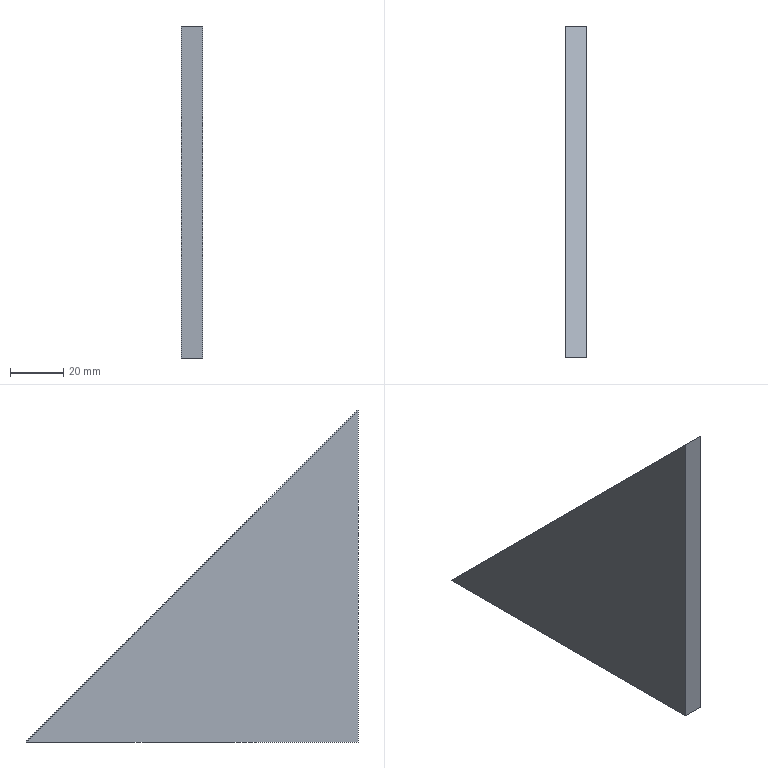Component | SolidWorks | 001ReinforcingRib-1 | 1 solid | 5 faces | box 8 x 125 x 125 mm | volume 62500 mm3 | plane 5 | material Plain Carbon Steel
build123d program:
from build123d import *

# Parameters (mm, degrees)
BOSS_EXTRUDE1_DEPTH = 8


with BuildPart() as part:
    # Sketch1 → Boss-Extrude1 (new body)
    with BuildSketch(Plane.XY):
        Polygon((0, 125), (0, 0), (125, 0), align=None)
    extrude(amount=BOSS_EXTRUDE1_DEPTH)


solid = part.part

# Placed as in the assembly
solid = solid.moved(Location((-37, 37, 0), (0, -90, 0)))
STEP:
#1=COLOUR_RGB('',0.7922,0.8196,0.9333);
#2=FILL_AREA_STYLE_COLOUR('',#1);
#3=FILL_AREA_STYLE('',(#2));
#4=SURFACE_STYLE_FILL_AREA(#3);
#5=SURFACE_SIDE_STYLE('',(#4));
#6=SURFACE_STYLE_USAGE(.BOTH.,#5);
#7=PRESENTATION_STYLE_ASSIGNMENT((#6));
#8=CARTESIAN_POINT('',(-1.457,1.457,4.921));
#9=VERTEX_POINT('',#8);
#10=CARTESIAN_POINT('',(-1.457,6.378,-0.));
#11=VERTEX_POINT('',#10);
#12=CARTESIAN_POINT('',(-1.457,1.457,4.921));
#13=DIRECTION('',(0.,0.7071,-0.7071));
#14=VECTOR('',#13,39.37);
#15=LINE('',#12,#14);
#16=EDGE_CURVE('',#9,#11,#15,.T.);
#17=ORIENTED_EDGE('',*,*,#16,.T.);
#18=CARTESIAN_POINT('',(-1.772,6.378,-0.));
#19=VERTEX_POINT('',#18);
#20=CARTESIAN_POINT('',(-1.772,6.378,-0.));
#21=DIRECTION('',(1.,0.,0.));
#22=VECTOR('',#21,39.37);
#23=LINE('',#20,#22);
#24=EDGE_CURVE('',#19,#11,#23,.T.);
#25=ORIENTED_EDGE('',*,*,#24,.F.);
#26=CARTESIAN_POINT('',(-1.772,1.457,4.921));
#27=VERTEX_POINT('',#26);
#28=CARTESIAN_POINT('',(-1.772,1.457,4.921));
#29=DIRECTION('',(0.,0.7071,-0.7071));
#30=VECTOR('',#29,39.37);
#31=LINE('',#28,#30);
#32=EDGE_CURVE('',#27,#19,#31,.T.);
#33=ORIENTED_EDGE('',*,*,#32,.F.);
#34=CARTESIAN_POINT('',(-1.772,1.457,4.921));
#35=DIRECTION('',(1.,0.,0.));
#36=VECTOR('',#35,39.37);
#37=LINE('',#34,#36);
#38=EDGE_CURVE('',#27,#9,#37,.T.);
#39=ORIENTED_EDGE('',*,*,#38,.T.);
#40=EDGE_LOOP('',(#17,#25,#33,#39));
#41=FACE_OUTER_BOUND('',#40,.T.);
#42=CARTESIAN_POINT('',(-1.772,1.457,4.921));
#43=DIRECTION('',(0.,-0.7071,-0.7071));
#44=DIRECTION('',(0.,-0.7071,0.7071));
#45=AXIS2_PLACEMENT_3D('',#42,#43,#44);
#46=PLANE('',#45);
#47=ADVANCED_FACE('',(#41),#46,.F.);
#48=CARTESIAN_POINT('',(-1.457,1.457,-0.));
#49=VERTEX_POINT('',#48);
#50=CARTESIAN_POINT('',(-1.457,6.378,-0.));
#51=DIRECTION('',(0.,-1.,-0.));
#52=VECTOR('',#51,39.37);
#53=LINE('',#50,#52);
#54=EDGE_CURVE('',#11,#49,#53,.T.);
#55=ORIENTED_EDGE('',*,*,#54,.T.);
#56=CARTESIAN_POINT('',(-1.772,1.457,-0.));
#57=VERTEX_POINT('',#56);
#58=CARTESIAN_POINT('',(-1.772,1.457,-0.));
#59=DIRECTION('',(1.,0.,0.));
#60=VECTOR('',#59,39.37);
#61=LINE('',#58,#60);
#62=EDGE_CURVE('',#57,#49,#61,.T.);
#63=ORIENTED_EDGE('',*,*,#62,.F.);
#64=CARTESIAN_POINT('',(-1.772,6.378,-0.));
#65=DIRECTION('',(0.,-1.,-0.));
#66=VECTOR('',#65,39.37);
#67=LINE('',#64,#66);
#68=EDGE_CURVE('',#19,#57,#67,.T.);
#69=ORIENTED_EDGE('',*,*,#68,.F.);
#70=ORIENTED_EDGE('',*,*,#24,.T.);
#71=EDGE_LOOP('',(#55,#63,#69,#70));
#72=FACE_OUTER_BOUND('',#71,.T.);
#73=CARTESIAN_POINT('',(-1.772,6.378,-0.));
#74=DIRECTION('',(0.,-0.,1.));
#75=DIRECTION('',(0.,1.,0.));
#76=AXIS2_PLACEMENT_3D('',#73,#74,#75);
#77=PLANE('',#76);
#78=ADVANCED_FACE('',(#72),#77,.F.);
#79=CARTESIAN_POINT('',(-1.457,1.457,-0.));
#80=DIRECTION('',(0.,0.,1.));
#81=VECTOR('',#80,39.37);
#82=LINE('',#79,#81);
#83=EDGE_CURVE('',#49,#9,#82,.T.);
#84=ORIENTED_EDGE('',*,*,#83,.T.);
#85=ORIENTED_EDGE('',*,*,#38,.F.);
#86=CARTESIAN_POINT('',(-1.772,1.457,-0.));
#87=DIRECTION('',(0.,0.,1.));
#88=VECTOR('',#87,39.37);
#89=LINE('',#86,#88);
#90=EDGE_CURVE('',#57,#27,#89,.T.);
#91=ORIENTED_EDGE('',*,*,#90,.F.);
#92=ORIENTED_EDGE('',*,*,#62,.T.);
#93=EDGE_LOOP('',(#84,#85,#91,#92));
#94=FACE_OUTER_BOUND('',#93,.T.);
#95=CARTESIAN_POINT('',(-1.772,1.457,-0.));
#96=DIRECTION('',(0.,1.,0.));
#97=DIRECTION('',(-1.,0.,0.));
#98=AXIS2_PLACEMENT_3D('',#95,#96,#97);
#99=PLANE('',#98);
#100=ADVANCED_FACE('',(#94),#99,.F.);
#101=ORIENTED_EDGE('',*,*,#32,.T.);
#102=ORIENTED_EDGE('',*,*,#68,.T.);
#103=ORIENTED_EDGE('',*,*,#90,.T.);
#104=EDGE_LOOP('',(#101,#102,#103));
#105=FACE_OUTER_BOUND('',#104,.T.);
#106=CARTESIAN_POINT('',(-1.772,6.378,-0.));
#107=DIRECTION('',(-1.,0.,0.));
#108=DIRECTION('',(0.,0.,1.));
#109=AXIS2_PLACEMENT_3D('',#106,#107,#108);
#110=PLANE('',#109);
#111=ADVANCED_FACE('',(#105),#110,.T.);
#112=ORIENTED_EDGE('',*,*,#16,.F.);
#113=ORIENTED_EDGE('',*,*,#83,.F.);
#114=ORIENTED_EDGE('',*,*,#54,.F.);
#115=EDGE_LOOP('',(#112,#113,#114));
#116=FACE_OUTER_BOUND('',#115,.T.);
#117=CARTESIAN_POINT('',(-1.457,6.378,-0.));
#118=DIRECTION('',(-1.,0.,0.));
#119=DIRECTION('',(0.,0.,1.));
#120=AXIS2_PLACEMENT_3D('',#117,#118,#119);
#121=PLANE('',#120);
#122=ADVANCED_FACE('',(#116),#121,.F.);
#123=CLOSED_SHELL('',(#47,#78,#100,#111,#122));
#124=MANIFOLD_SOLID_BREP('',#123);
#125=STYLED_ITEM('',(#7),#124);
#126=PRESENTATION_LAYER_ASSIGNMENT('','',(#125));
#127=CARTESIAN_POINT('',(0.,0.,0.));
#128=DIRECTION('',(0.,0.,1.));
#129=DIRECTION('',(1.,0.,0.));
#130=AXIS2_PLACEMENT_3D('',#127,#128,#129);
#131=(LENGTH_UNIT()NAMED_UNIT(*)SI_UNIT($,.METRE.));
#132=LENGTH_MEASURE_WITH_UNIT(LENGTH_MEASURE(0.0254),#131);
#133=DIMENSIONAL_EXPONENTS(1.,0.,0.,0.,0.,0.,0.);
#134=(CONVERSION_BASED_UNIT('',#132)LENGTH_UNIT()NAMED_UNIT(#133));
#135=UNCERTAINTY_MEASURE_WITH_UNIT(LENGTH_MEASURE(0.00001),#134,'','');
#136=(NAMED_UNIT(*)PLANE_ANGLE_UNIT()SI_UNIT($,.RADIAN.));
#137=(NAMED_UNIT(*)SI_UNIT($,.STERADIAN.)SOLID_ANGLE_UNIT());
#138=(GEOMETRIC_REPRESENTATION_CONTEXT(3)GLOBAL_UNCERTAINTY_ASSIGNED_CONTEXT((#135))GLOBAL_UNIT_ASSIGNED_CONTEXT((#134,#136,#137))REPRESENTATION_CONTEXT('',''));
#139=ADVANCED_BREP_SHAPE_REPRESENTATION('',(#124,#130),#138);
#140=(LENGTH_UNIT()NAMED_UNIT(*)SI_UNIT($,.METRE.));
#141=LENGTH_MEASURE_WITH_UNIT(LENGTH_MEASURE(0.0254),#140);
#142=DIMENSIONAL_EXPONENTS(1.,0.,0.,0.,0.,0.,0.);
#143=(CONVERSION_BASED_UNIT('',#141)LENGTH_UNIT()NAMED_UNIT(#142));
#144=UNCERTAINTY_MEASURE_WITH_UNIT(LENGTH_MEASURE(0.00001),#143,'','');
#145=(NAMED_UNIT(*)PLANE_ANGLE_UNIT()SI_UNIT($,.RADIAN.));
#146=(NAMED_UNIT(*)SI_UNIT($,.STERADIAN.)SOLID_ANGLE_UNIT());
#147=(GEOMETRIC_REPRESENTATION_CONTEXT(3)GLOBAL_UNCERTAINTY_ASSIGNED_CONTEXT((#144))GLOBAL_UNIT_ASSIGNED_CONTEXT((#143,#145,#146))REPRESENTATION_CONTEXT('',''));
#148=MECHANICAL_DESIGN_GEOMETRIC_PRESENTATION_REPRESENTATION('',(#125),#147);